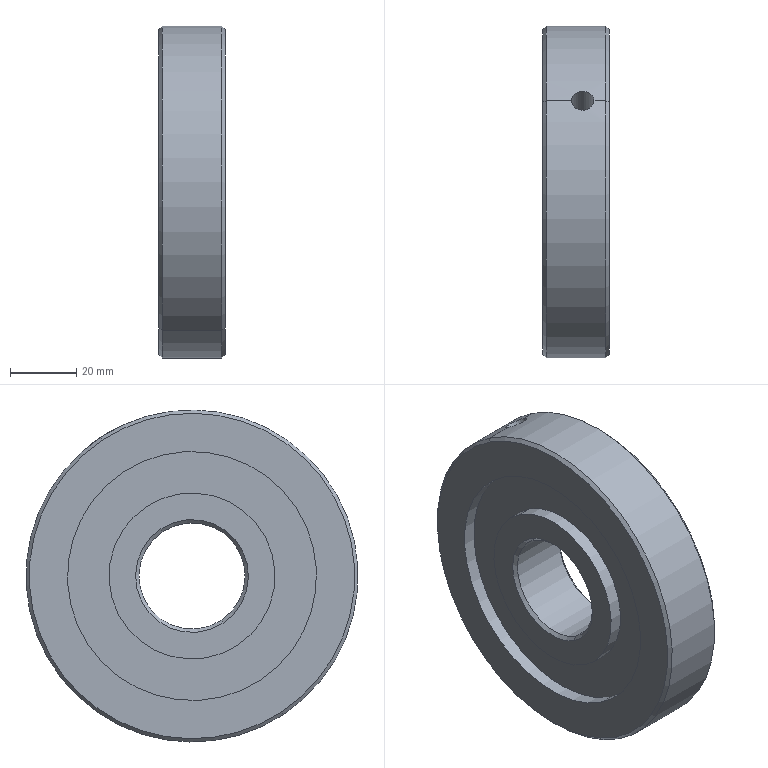Component | SolidWorks | Flange2-1 | 1 solid | 22 faces | box 20 x 100 x 100 mm | volume 129525 mm3 | cylinder 10 | cone 8 | plane 4 | commonest cylinder face diameters 6.8 x2 50 x2 75 x2 32 x2 100 x2
build123d program:
from build123d import *

# Parameters (mm, degrees)
SKETCH1_R             = 50
SKETCH1_R_2           = 16
BOSS_EXTRUDE1_DEPTH   = 20
CHAMFER1_SIZE         = 1
SKETCH2_R             = 37.5
SKETCH2_R_2           = 25
CUT_EXTRUDE1_DEPTH    = 4
M8_TAPPED_HOLE1_D     = 6.8
M8_TAPPED_HOLE1_DEPTH = 41.75
M8_TAPPED_HOLE1_TIP   = 2.043


with BuildPart() as part:
    # Sketch1 → Boss-Extrude1 (new body)
    with BuildSketch(Plane.XY):
        Circle(SKETCH1_R)
        Circle(SKETCH1_R_2, mode=Mode.SUBTRACT)
    extrude(amount=BOSS_EXTRUDE1_DEPTH)

    # Chamfer1
    chamfer1_edges = [part.edges().sort_by_distance(p)[0] for p in [
        (-50, 0, 0),
        (-50, 0, 20),
        (-16, 0, 0),
        (-16, 0, 20),
    ]]
    chamfer(chamfer1_edges, length=CHAMFER1_SIZE)

    # Sketch2 → Cut-Extrude1 (cut)
    with BuildSketch(Plane.XY.offset(20)):
        Circle(SKETCH2_R)
        Circle(SKETCH2_R_2, mode=Mode.SUBTRACT)
    extrude(amount=-CUT_EXTRUDE1_DEPTH, mode=Mode.SUBTRACT)

    # M8 Tapped Hole1
    with Locations(Plane(origin=(50, 0, 8), x_dir=(0, 1, 0), z_dir=(1, 0, 0))):
        with Locations((0, 0)):
            Hole(M8_TAPPED_HOLE1_D / 2, depth=M8_TAPPED_HOLE1_DEPTH)
            with Locations((0, 0, -(M8_TAPPED_HOLE1_DEPTH + M8_TAPPED_HOLE1_TIP / 2))):  # 118° drill point
                Cone(0, M8_TAPPED_HOLE1_D / 2, M8_TAPPED_HOLE1_TIP, mode=Mode.SUBTRACT)


solid = part.part

# Placed as in the assembly
solid = solid.moved(Location((-136.809, -4.181, 0), (-33.315, -90, 0)))
STEP:
#1=COLOUR_RGB('',0.7922,0.8196,0.9333);
#2=FILL_AREA_STYLE_COLOUR('',#1);
#3=FILL_AREA_STYLE('',(#2));
#4=SURFACE_STYLE_FILL_AREA(#3);
#5=SURFACE_SIDE_STYLE('',(#4));
#6=SURFACE_STYLE_USAGE(.BOTH.,#5);
#7=PRESENTATION_STYLE_ASSIGNMENT((#6));
#8=CARTESIAN_POINT('',(-5.567,0.1814,0.5264));
#9=VERTEX_POINT('',#8);
#10=CARTESIAN_POINT('',(-5.835,0.1814,0.5264));
#11=VERTEX_POINT('',#10);
#12=CARTESIAN_POINT('',(-5.567,0.1814,0.5264));
#13=CARTESIAN_POINT('',(-5.567,0.174,0.5313));
#14=CARTESIAN_POINT('',(-5.568,0.1666,0.5359));
#15=CARTESIAN_POINT('',(-5.572,0.1518,0.5447));
#16=CARTESIAN_POINT('',(-5.574,0.1444,0.549));
#17=CARTESIAN_POINT('',(-5.581,0.1302,0.5568));
#18=CARTESIAN_POINT('',(-5.585,0.1233,0.5603));
#19=CARTESIAN_POINT('',(-5.595,0.1102,0.5669));
#20=CARTESIAN_POINT('',(-5.6,0.104,0.5698));
#21=CARTESIAN_POINT('',(-5.613,0.09266,0.575));
#22=CARTESIAN_POINT('',(-5.619,0.08753,0.5773));
#23=CARTESIAN_POINT('',(-5.634,0.07839,0.5812));
#24=CARTESIAN_POINT('',(-5.642,0.07449,0.5828));
#25=CARTESIAN_POINT('',(-5.658,0.06817,0.5853));
#26=CARTESIAN_POINT('',(-5.666,0.06571,0.5863));
#27=CARTESIAN_POINT('',(-5.684,0.06243,0.5876));
#28=CARTESIAN_POINT('',(-5.692,0.06161,0.5879));
#29=CARTESIAN_POINT('',(-5.71,0.0616,0.5879));
#30=CARTESIAN_POINT('',(-5.719,0.06244,0.5876));
#31=CARTESIAN_POINT('',(-5.736,0.06571,0.5863));
#32=CARTESIAN_POINT('',(-5.744,0.06812,0.5854));
#33=CARTESIAN_POINT('',(-5.761,0.07449,0.5828));
#34=CARTESIAN_POINT('',(-5.768,0.07843,0.5812));
#35=CARTESIAN_POINT('',(-5.783,0.08747,0.5773));
#36=CARTESIAN_POINT('',(-5.79,0.09264,0.575));
#37=CARTESIAN_POINT('',(-5.802,0.1041,0.5698));
#38=CARTESIAN_POINT('',(-5.808,0.1102,0.5669));
#39=CARTESIAN_POINT('',(-5.817,0.1232,0.5604));
#40=CARTESIAN_POINT('',(-5.821,0.1302,0.5567));
#41=CARTESIAN_POINT('',(-5.828,0.1445,0.5489));
#42=CARTESIAN_POINT('',(-5.831,0.1517,0.5448));
#43=CARTESIAN_POINT('',(-5.834,0.1665,0.5359));
#44=CARTESIAN_POINT('',(-5.835,0.1741,0.5312));
#45=CARTESIAN_POINT('',(-5.835,0.1814,0.5264));
#46=B_SPLINE_CURVE_WITH_KNOTS('',3,(#12,#13,#14,#15,#16,#17,#18,#19,#20,#21,#22,#23,#24,#25,#26,#27,#28,#29,#30,#31,#32,#33,#34,#35,#36,#37,#38,#39,#40,#41,#42,#43,#44,#45),.UNSPECIFIED.,.F.,.F.,(4,2,2,2,2,2,2,2,2,2,2,2,2,2,2,2,4),(0.,0.0006663,0.001333,0.001999,0.002665,0.003331,0.003998,0.004664,0.00533,0.005996,0.006663,0.007329,0.007995,0.008662,0.009328,0.009994,0.01066),.UNSPECIFIED.);
#47=EDGE_CURVE('',#9,#11,#46,.T.);
#48=ORIENTED_EDGE('',*,*,#47,.T.);
#49=CARTESIAN_POINT('',(-5.835,0.9166,1.645));
#50=VERTEX_POINT('',#49);
#51=CARTESIAN_POINT('',(-5.835,0.9166,1.645));
#52=DIRECTION('',(-0.,0.5492,0.8357));
#53=VECTOR('',#52,39.37);
#54=LINE('',#51,#53);
#55=EDGE_CURVE('',#11,#50,#54,.T.);
#56=ORIENTED_EDGE('',*,*,#55,.T.);
#57=CARTESIAN_POINT('',(-5.567,0.9166,1.645));
#58=VERTEX_POINT('',#57);
#59=CARTESIAN_POINT('',(-5.567,0.9166,1.645));
#60=CARTESIAN_POINT('',(-5.567,0.9092,1.65));
#61=CARTESIAN_POINT('',(-5.568,0.9019,1.655));
#62=CARTESIAN_POINT('',(-5.572,0.8874,1.664));
#63=CARTESIAN_POINT('',(-5.574,0.8802,1.668));
#64=CARTESIAN_POINT('',(-5.581,0.8665,1.677));
#65=CARTESIAN_POINT('',(-5.585,0.8599,1.681));
#66=CARTESIAN_POINT('',(-5.595,0.8474,1.688));
#67=CARTESIAN_POINT('',(-5.6,0.8415,1.692));
#68=CARTESIAN_POINT('',(-5.613,0.8309,1.698));
#69=CARTESIAN_POINT('',(-5.619,0.8261,1.701));
#70=CARTESIAN_POINT('',(-5.634,0.8176,1.706));
#71=CARTESIAN_POINT('',(-5.642,0.814,1.708));
#72=CARTESIAN_POINT('',(-5.658,0.8082,1.711));
#73=CARTESIAN_POINT('',(-5.666,0.8059,1.713));
#74=CARTESIAN_POINT('',(-5.684,0.8029,1.714));
#75=CARTESIAN_POINT('',(-5.692,0.8022,1.715));
#76=CARTESIAN_POINT('',(-5.71,0.8022,1.715));
#77=CARTESIAN_POINT('',(-5.719,0.803,1.714));
#78=CARTESIAN_POINT('',(-5.736,0.8059,1.713));
#79=CARTESIAN_POINT('',(-5.744,0.8081,1.711));
#80=CARTESIAN_POINT('',(-5.76,0.814,1.708));
#81=CARTESIAN_POINT('',(-5.768,0.8176,1.706));
#82=CARTESIAN_POINT('',(-5.783,0.826,1.701));
#83=CARTESIAN_POINT('',(-5.79,0.8308,1.698));
#84=CARTESIAN_POINT('',(-5.802,0.8416,1.692));
#85=CARTESIAN_POINT('',(-5.808,0.8474,1.688));
#86=CARTESIAN_POINT('',(-5.817,0.8598,1.681));
#87=CARTESIAN_POINT('',(-5.821,0.8665,1.677));
#88=CARTESIAN_POINT('',(-5.828,0.8803,1.668));
#89=CARTESIAN_POINT('',(-5.831,0.8874,1.664));
#90=CARTESIAN_POINT('',(-5.834,0.9018,1.655));
#91=CARTESIAN_POINT('',(-5.835,0.9093,1.65));
#92=CARTESIAN_POINT('',(-5.835,0.9166,1.645));
#93=B_SPLINE_CURVE_WITH_KNOTS('',3,(#59,#60,#61,#62,#63,#64,#65,#66,#67,#68,#69,#70,#71,#72,#73,#74,#75,#76,#77,#78,#79,#80,#81,#82,#83,#84,#85,#86,#87,#88,#89,#90,#91,#92),.UNSPECIFIED.,.F.,.F.,(4,2,2,2,2,2,2,2,2,2,2,2,2,2,2,2,4),(0.,0.0006646,0.001329,0.001994,0.002658,0.003323,0.003987,0.004652,0.005317,0.005981,0.006646,0.00731,0.007975,0.008639,0.009304,0.009968,0.01063),.UNSPECIFIED.);
#94=EDGE_CURVE('',#58,#50,#93,.T.);
#95=ORIENTED_EDGE('',*,*,#94,.F.);
#96=CARTESIAN_POINT('',(-5.567,0.9166,1.645));
#97=DIRECTION('',(-0.,0.5492,0.8357));
#98=VECTOR('',#97,39.37);
#99=LINE('',#96,#98);
#100=EDGE_CURVE('',#9,#58,#99,.T.);
#101=ORIENTED_EDGE('',*,*,#100,.F.);
#102=EDGE_LOOP('',(#48,#56,#95,#101));
#103=FACE_OUTER_BOUND('',#102,.T.);
#104=CARTESIAN_POINT('',(-5.701,0.9166,1.645));
#105=DIRECTION('',(-0.,0.5492,0.8357));
#106=DIRECTION('',(1.,0.,0.));
#107=AXIS2_PLACEMENT_3D('',#104,#105,#106);
#108=CYLINDRICAL_SURFACE('',#107,0.1339);
#109=ADVANCED_FACE('',(#103),#108,.F.);
#110=CARTESIAN_POINT('',(-6.016,0.376,0.8225));
#111=VERTEX_POINT('',#110);
#112=CARTESIAN_POINT('',(-6.016,-0.7052,-0.8225));
#113=VERTEX_POINT('',#112);
#114=CARTESIAN_POINT('',(-6.016,-0.1646,-0.));
#115=DIRECTION('',(-1.,-0.,-0.));
#116=DIRECTION('',(0.,0.5492,0.8357));
#117=AXIS2_PLACEMENT_3D('',#114,#115,#116);
#118=CIRCLE('',#117,0.9843);
#119=EDGE_CURVE('',#111,#113,#118,.T.);
#120=ORIENTED_EDGE('',*,*,#119,.T.);
#121=CARTESIAN_POINT('',(-6.174,-0.7052,-0.8225));
#122=VERTEX_POINT('',#121);
#123=CARTESIAN_POINT('',(-6.016,-0.7052,-0.8225));
#124=DIRECTION('',(-1.,-0.,-0.));
#125=VECTOR('',#124,39.37);
#126=LINE('',#123,#125);
#127=EDGE_CURVE('',#113,#122,#126,.T.);
#128=ORIENTED_EDGE('',*,*,#127,.T.);
#129=CARTESIAN_POINT('',(-6.174,0.376,0.8225));
#130=VERTEX_POINT('',#129);
#131=CARTESIAN_POINT('',(-6.174,-0.1646,-0.));
#132=DIRECTION('',(-1.,-0.,-0.));
#133=DIRECTION('',(0.,0.5492,0.8357));
#134=AXIS2_PLACEMENT_3D('',#131,#132,#133);
#135=CIRCLE('',#134,0.9843);
#136=EDGE_CURVE('',#130,#122,#135,.T.);
#137=ORIENTED_EDGE('',*,*,#136,.F.);
#138=CARTESIAN_POINT('',(-6.016,0.376,0.8225));
#139=DIRECTION('',(-1.,-0.,-0.));
#140=VECTOR('',#139,39.37);
#141=LINE('',#138,#140);
#142=EDGE_CURVE('',#111,#130,#141,.T.);
#143=ORIENTED_EDGE('',*,*,#142,.F.);
#144=EDGE_LOOP('',(#120,#128,#137,#143));
#145=FACE_OUTER_BOUND('',#144,.T.);
#146=CARTESIAN_POINT('',(-6.016,-0.1646,-0.));
#147=DIRECTION('',(-1.,-0.,-0.));
#148=DIRECTION('',(0.,0.5492,0.8357));
#149=AXIS2_PLACEMENT_3D('',#146,#147,#148);
#150=CYLINDRICAL_SURFACE('',#149,0.9843);
#151=ADVANCED_FACE('',(#145),#150,.T.);
#152=CARTESIAN_POINT('',(-6.016,-0.9755,-1.234));
#153=VERTEX_POINT('',#152);
#154=CARTESIAN_POINT('',(-6.016,0.6463,1.234));
#155=VERTEX_POINT('',#154);
#156=CARTESIAN_POINT('',(-6.016,-0.1646,-0.));
#157=DIRECTION('',(-1.,-0.,-0.));
#158=DIRECTION('',(0.,0.5492,0.8357));
#159=AXIS2_PLACEMENT_3D('',#156,#157,#158);
#160=CIRCLE('',#159,1.476);
#161=EDGE_CURVE('',#153,#155,#160,.T.);
#162=ORIENTED_EDGE('',*,*,#161,.F.);
#163=CARTESIAN_POINT('',(-6.174,-0.9755,-1.234));
#164=VERTEX_POINT('',#163);
#165=CARTESIAN_POINT('',(-6.016,-0.9755,-1.234));
#166=DIRECTION('',(-1.,-0.,-0.));
#167=VECTOR('',#166,39.37);
#168=LINE('',#165,#167);
#169=EDGE_CURVE('',#153,#164,#168,.T.);
#170=ORIENTED_EDGE('',*,*,#169,.T.);
#171=CARTESIAN_POINT('',(-6.174,0.6463,1.234));
#172=VERTEX_POINT('',#171);
#173=CARTESIAN_POINT('',(-6.174,-0.1646,-0.));
#174=DIRECTION('',(-1.,-0.,-0.));
#175=DIRECTION('',(0.,0.5492,0.8357));
#176=AXIS2_PLACEMENT_3D('',#173,#174,#175);
#177=CIRCLE('',#176,1.476);
#178=EDGE_CURVE('',#164,#172,#177,.T.);
#179=ORIENTED_EDGE('',*,*,#178,.T.);
#180=CARTESIAN_POINT('',(-6.016,0.6463,1.234));
#181=DIRECTION('',(-1.,-0.,-0.));
#182=VECTOR('',#181,39.37);
#183=LINE('',#180,#182);
#184=EDGE_CURVE('',#155,#172,#183,.T.);
#185=ORIENTED_EDGE('',*,*,#184,.F.);
#186=EDGE_LOOP('',(#162,#170,#179,#185));
#187=FACE_OUTER_BOUND('',#186,.T.);
#188=CARTESIAN_POINT('',(-6.016,-0.1646,-0.));
#189=DIRECTION('',(-1.,-0.,-0.));
#190=DIRECTION('',(0.,0.5492,0.8357));
#191=AXIS2_PLACEMENT_3D('',#188,#189,#190);
#192=CYLINDRICAL_SURFACE('',#191,1.476);
#193=ADVANCED_FACE('',(#187),#192,.F.);
#194=CARTESIAN_POINT('',(-6.174,0.8949,1.612));
#195=VERTEX_POINT('',#194);
#196=CARTESIAN_POINT('',(-6.174,-1.224,-1.612));
#197=VERTEX_POINT('',#196);
#198=CARTESIAN_POINT('',(-6.174,-0.1646,-0.));
#199=DIRECTION('',(-1.,-0.,-0.));
#200=DIRECTION('',(0.,0.5492,0.8357));
#201=AXIS2_PLACEMENT_3D('',#198,#199,#200);
#202=CIRCLE('',#201,1.929);
#203=EDGE_CURVE('',#195,#197,#202,.T.);
#204=ORIENTED_EDGE('',*,*,#203,.F.);
#205=CARTESIAN_POINT('',(-6.134,0.9166,1.645));
#206=VERTEX_POINT('',#205);
#207=CARTESIAN_POINT('',(-6.174,0.8949,1.612));
#208=DIRECTION('',(0.7071,0.3884,0.5909));
#209=VECTOR('',#208,39.37);
#210=LINE('',#207,#209);
#211=EDGE_CURVE('',#195,#206,#210,.T.);
#212=ORIENTED_EDGE('',*,*,#211,.T.);
#213=CARTESIAN_POINT('',(-6.134,-1.246,-1.645));
#214=VERTEX_POINT('',#213);
#215=CARTESIAN_POINT('',(-6.134,-0.1646,-0.));
#216=DIRECTION('',(1.,0.,0.));
#217=DIRECTION('',(0.,0.5492,0.8357));
#218=AXIS2_PLACEMENT_3D('',#215,#216,#217);
#219=CIRCLE('',#218,1.969);
#220=EDGE_CURVE('',#214,#206,#219,.T.);
#221=ORIENTED_EDGE('',*,*,#220,.F.);
#222=CARTESIAN_POINT('',(-6.174,-1.224,-1.612));
#223=DIRECTION('',(0.7071,-0.3884,-0.5909));
#224=VECTOR('',#223,39.37);
#225=LINE('',#222,#224);
#226=EDGE_CURVE('',#197,#214,#225,.T.);
#227=ORIENTED_EDGE('',*,*,#226,.F.);
#228=EDGE_LOOP('',(#204,#212,#221,#227));
#229=FACE_OUTER_BOUND('',#228,.T.);
#230=CARTESIAN_POINT('',(-6.174,-0.1646,-0.));
#231=DIRECTION('',(1.,0.,0.));
#232=DIRECTION('',(0.,-0.5492,-0.8357));
#233=AXIS2_PLACEMENT_3D('',#230,#231,#232);
#234=CONICAL_SURFACE('',#233,1.929,0.7854);
#235=ADVANCED_FACE('',(#229),#234,.T.);
#236=CARTESIAN_POINT('',(-6.134,-0.5106,-0.5264));
#237=VERTEX_POINT('',#236);
#238=CARTESIAN_POINT('',(-6.134,0.1814,0.5264));
#239=VERTEX_POINT('',#238);
#240=CARTESIAN_POINT('',(-6.134,-0.1646,-0.));
#241=DIRECTION('',(-1.,-0.,-0.));
#242=DIRECTION('',(0.,0.5492,0.8357));
#243=AXIS2_PLACEMENT_3D('',#240,#241,#242);
#244=CIRCLE('',#243,0.6299);
#245=EDGE_CURVE('',#237,#239,#244,.T.);
#246=ORIENTED_EDGE('',*,*,#245,.F.);
#247=CARTESIAN_POINT('',(-6.174,-0.5322,-0.5593));
#248=VERTEX_POINT('',#247);
#249=CARTESIAN_POINT('',(-6.134,-0.5106,-0.5264));
#250=DIRECTION('',(-0.7071,-0.3884,-0.5909));
#251=VECTOR('',#250,39.37);
#252=LINE('',#249,#251);
#253=EDGE_CURVE('',#237,#248,#252,.T.);
#254=ORIENTED_EDGE('',*,*,#253,.T.);
#255=CARTESIAN_POINT('',(-6.174,0.203,0.5593));
#256=VERTEX_POINT('',#255);
#257=CARTESIAN_POINT('',(-6.174,-0.1646,-0.));
#258=DIRECTION('',(1.,0.,0.));
#259=DIRECTION('',(0.,0.5492,0.8357));
#260=AXIS2_PLACEMENT_3D('',#257,#258,#259);
#261=CIRCLE('',#260,0.6693);
#262=EDGE_CURVE('',#256,#248,#261,.T.);
#263=ORIENTED_EDGE('',*,*,#262,.F.);
#264=CARTESIAN_POINT('',(-6.134,0.1814,0.5264));
#265=DIRECTION('',(-0.7071,0.3884,0.5909));
#266=VECTOR('',#265,39.37);
#267=LINE('',#264,#266);
#268=EDGE_CURVE('',#239,#256,#267,.T.);
#269=ORIENTED_EDGE('',*,*,#268,.F.);
#270=EDGE_LOOP('',(#246,#254,#263,#269));
#271=FACE_OUTER_BOUND('',#270,.T.);
#272=CARTESIAN_POINT('',(-6.134,-0.1646,-0.));
#273=DIRECTION('',(-1.,-0.,-0.));
#274=DIRECTION('',(0.,0.5492,0.8357));
#275=AXIS2_PLACEMENT_3D('',#272,#273,#274);
#276=CONICAL_SURFACE('',#275,0.6299,0.7854);
#277=ADVANCED_FACE('',(#271),#276,.F.);
#278=CARTESIAN_POINT('',(-5.386,-1.224,-1.612));
#279=VERTEX_POINT('',#278);
#280=CARTESIAN_POINT('',(-5.386,0.8949,1.612));
#281=VERTEX_POINT('',#280);
#282=CARTESIAN_POINT('',(-5.386,-0.1646,0.));
#283=DIRECTION('',(1.,0.,0.));
#284=DIRECTION('',(0.,0.5492,0.8357));
#285=AXIS2_PLACEMENT_3D('',#282,#283,#284);
#286=CIRCLE('',#285,1.929);
#287=EDGE_CURVE('',#279,#281,#286,.T.);
#288=ORIENTED_EDGE('',*,*,#287,.F.);
#289=CARTESIAN_POINT('',(-5.426,-1.246,-1.645));
#290=VERTEX_POINT('',#289);
#291=CARTESIAN_POINT('',(-5.426,-1.246,-1.645));
#292=DIRECTION('',(-0.7071,-0.3884,-0.5909));
#293=VECTOR('',#292,39.37);
#294=LINE('',#291,#293);
#295=EDGE_CURVE('',#279,#290,#294,.T.);
#296=ORIENTED_EDGE('',*,*,#295,.T.);
#297=CARTESIAN_POINT('',(-5.426,0.9166,1.645));
#298=VERTEX_POINT('',#297);
#299=CARTESIAN_POINT('',(-5.426,-0.1646,0.));
#300=DIRECTION('',(-1.,-0.,-0.));
#301=DIRECTION('',(0.,0.5492,0.8357));
#302=AXIS2_PLACEMENT_3D('',#299,#300,#301);
#303=CIRCLE('',#302,1.969);
#304=EDGE_CURVE('',#298,#290,#303,.T.);
#305=ORIENTED_EDGE('',*,*,#304,.F.);
#306=CARTESIAN_POINT('',(-5.426,0.9166,1.645));
#307=DIRECTION('',(-0.7071,0.3884,0.5909));
#308=VECTOR('',#307,39.37);
#309=LINE('',#306,#308);
#310=EDGE_CURVE('',#281,#298,#309,.T.);
#311=ORIENTED_EDGE('',*,*,#310,.F.);
#312=EDGE_LOOP('',(#288,#296,#305,#311));
#313=FACE_OUTER_BOUND('',#312,.T.);
#314=CARTESIAN_POINT('',(-5.426,-0.1646,0.));
#315=DIRECTION('',(-1.,-0.,-0.));
#316=DIRECTION('',(0.,0.5492,0.8357));
#317=AXIS2_PLACEMENT_3D('',#314,#315,#316);
#318=CONICAL_SURFACE('',#317,1.969,0.7854);
#319=ADVANCED_FACE('',(#313),#318,.T.);
#320=CARTESIAN_POINT('',(-5.426,0.1814,0.5264));
#321=VERTEX_POINT('',#320);
#322=CARTESIAN_POINT('',(-5.426,-0.5106,-0.5264));
#323=VERTEX_POINT('',#322);
#324=CARTESIAN_POINT('',(-5.426,-0.1646,0.));
#325=DIRECTION('',(1.,0.,0.));
#326=DIRECTION('',(0.,0.5492,0.8357));
#327=AXIS2_PLACEMENT_3D('',#324,#325,#326);
#328=CIRCLE('',#327,0.6299);
#329=EDGE_CURVE('',#321,#323,#328,.T.);
#330=ORIENTED_EDGE('',*,*,#329,.F.);
#331=CARTESIAN_POINT('',(-5.386,0.203,0.5593));
#332=VERTEX_POINT('',#331);
#333=CARTESIAN_POINT('',(-5.386,0.203,0.5593));
#334=DIRECTION('',(0.7071,0.3884,0.5909));
#335=VECTOR('',#334,39.37);
#336=LINE('',#333,#335);
#337=EDGE_CURVE('',#321,#332,#336,.T.);
#338=ORIENTED_EDGE('',*,*,#337,.T.);
#339=CARTESIAN_POINT('',(-5.386,-0.5322,-0.5593));
#340=VERTEX_POINT('',#339);
#341=CARTESIAN_POINT('',(-5.386,-0.1646,0.));
#342=DIRECTION('',(-1.,-0.,-0.));
#343=DIRECTION('',(0.,0.5492,0.8357));
#344=AXIS2_PLACEMENT_3D('',#341,#342,#343);
#345=CIRCLE('',#344,0.6693);
#346=EDGE_CURVE('',#340,#332,#345,.T.);
#347=ORIENTED_EDGE('',*,*,#346,.F.);
#348=CARTESIAN_POINT('',(-5.386,-0.5322,-0.5593));
#349=DIRECTION('',(0.7071,-0.3884,-0.5909));
#350=VECTOR('',#349,39.37);
#351=LINE('',#348,#350);
#352=EDGE_CURVE('',#323,#340,#351,.T.);
#353=ORIENTED_EDGE('',*,*,#352,.F.);
#354=EDGE_LOOP('',(#330,#338,#347,#353));
#355=FACE_OUTER_BOUND('',#354,.T.);
#356=CARTESIAN_POINT('',(-5.386,-0.1646,0.));
#357=DIRECTION('',(1.,0.,0.));
#358=DIRECTION('',(0.,-0.5492,-0.8357));
#359=AXIS2_PLACEMENT_3D('',#356,#357,#358);
#360=CONICAL_SURFACE('',#359,0.6693,0.7854);
#361=ADVANCED_FACE('',(#355),#360,.F.);
#362=ORIENTED_EDGE('',*,*,#245,.T.);
#363=CARTESIAN_POINT('',(-6.174,0.1814,0.5264));
#364=DIRECTION('',(1.,0.,0.));
#365=VECTOR('',#364,39.37);
#366=LINE('',#363,#365);
#367=EDGE_CURVE('',#239,#11,#366,.T.);
#368=ORIENTED_EDGE('',*,*,#367,.T.);
#369=ORIENTED_EDGE('',*,*,#47,.F.);
#370=CARTESIAN_POINT('',(-6.174,0.1814,0.5264));
#371=DIRECTION('',(1.,0.,0.));
#372=VECTOR('',#371,39.37);
#373=LINE('',#370,#372);
#374=EDGE_CURVE('',#9,#321,#373,.T.);
#375=ORIENTED_EDGE('',*,*,#374,.T.);
#376=ORIENTED_EDGE('',*,*,#329,.T.);
#377=CARTESIAN_POINT('',(-6.174,-0.5106,-0.5264));
#378=DIRECTION('',(1.,0.,0.));
#379=VECTOR('',#378,39.37);
#380=LINE('',#377,#379);
#381=EDGE_CURVE('',#237,#323,#380,.T.);
#382=ORIENTED_EDGE('',*,*,#381,.F.);
#383=EDGE_LOOP('',(#362,#368,#369,#375,#376,#382));
#384=FACE_OUTER_BOUND('',#383,.T.);
#385=CARTESIAN_POINT('',(-6.174,-0.1646,-0.));
#386=DIRECTION('',(1.,0.,0.));
#387=DIRECTION('',(0.,-0.5492,-0.8357));
#388=AXIS2_PLACEMENT_3D('',#385,#386,#387);
#389=CYLINDRICAL_SURFACE('',#388,0.6299);
#390=ADVANCED_FACE('',(#384),#389,.F.);
#391=ORIENTED_EDGE('',*,*,#220,.T.);
#392=CARTESIAN_POINT('',(-6.174,0.9166,1.645));
#393=DIRECTION('',(1.,0.,0.));
#394=VECTOR('',#393,39.37);
#395=LINE('',#392,#394);
#396=EDGE_CURVE('',#206,#50,#395,.T.);
#397=ORIENTED_EDGE('',*,*,#396,.T.);
#398=CARTESIAN_POINT('',(-5.835,0.9166,1.645));
#399=CARTESIAN_POINT('',(-5.835,0.9239,1.64));
#400=CARTESIAN_POINT('',(-5.834,0.9311,1.635));
#401=CARTESIAN_POINT('',(-5.831,0.9454,1.626));
#402=CARTESIAN_POINT('',(-5.828,0.9524,1.621));
#403=CARTESIAN_POINT('',(-5.821,0.9656,1.612));
#404=CARTESIAN_POINT('',(-5.817,0.972,1.607));
#405=CARTESIAN_POINT('',(-5.808,0.9839,1.599));
#406=CARTESIAN_POINT('',(-5.802,0.9894,1.595));
#407=CARTESIAN_POINT('',(-5.79,0.9994,1.588));
#408=CARTESIAN_POINT('',(-5.783,1.004,1.584));
#409=CARTESIAN_POINT('',(-5.768,1.012,1.578));
#410=CARTESIAN_POINT('',(-5.761,1.015,1.576));
#411=CARTESIAN_POINT('',(-5.744,1.02,1.572));
#412=CARTESIAN_POINT('',(-5.736,1.022,1.57));
#413=CARTESIAN_POINT('',(-5.719,1.025,1.568));
#414=CARTESIAN_POINT('',(-5.71,1.026,1.568));
#415=CARTESIAN_POINT('',(-5.692,1.026,1.568));
#416=CARTESIAN_POINT('',(-5.684,1.025,1.568));
#417=CARTESIAN_POINT('',(-5.667,1.023,1.57));
#418=CARTESIAN_POINT('',(-5.658,1.02,1.572));
#419=CARTESIAN_POINT('',(-5.642,1.015,1.576));
#420=CARTESIAN_POINT('',(-5.634,1.012,1.578));
#421=CARTESIAN_POINT('',(-5.62,1.004,1.584));
#422=CARTESIAN_POINT('',(-5.613,0.9995,1.587));
#423=CARTESIAN_POINT('',(-5.6,0.9895,1.595));
#424=CARTESIAN_POINT('',(-5.595,0.984,1.599));
#425=CARTESIAN_POINT('',(-5.585,0.9721,1.607));
#426=CARTESIAN_POINT('',(-5.581,0.9657,1.612));
#427=CARTESIAN_POINT('',(-5.571,0.9459,1.625));
#428=CARTESIAN_POINT('',(-5.567,0.9313,1.635));
#429=CARTESIAN_POINT('',(-5.567,0.9166,1.645));
#430=B_SPLINE_CURVE_WITH_KNOTS('',3,(#398,#399,#400,#401,#402,#403,#404,#405,#406,#407,#408,#409,#410,#411,#412,#413,#414,#415,#416,#417,#418,#419,#420,#421,#422,#423,#424,#425,#426,#427,#428,#429),.UNSPECIFIED.,.F.,.F.,(4,2,2,2,2,2,2,2,2,2,2,2,2,2,2,4),(0.01063,0.0113,0.01196,0.01263,0.01329,0.01396,0.01462,0.01528,0.01595,0.01661,0.01728,0.01794,0.01861,0.01927,0.01993,0.02126),.UNSPECIFIED.);
#431=EDGE_CURVE('',#50,#58,#430,.T.);
#432=ORIENTED_EDGE('',*,*,#431,.T.);
#433=CARTESIAN_POINT('',(-6.174,0.9166,1.645));
#434=DIRECTION('',(1.,0.,0.));
#435=VECTOR('',#434,39.37);
#436=LINE('',#433,#435);
#437=EDGE_CURVE('',#58,#298,#436,.T.);
#438=ORIENTED_EDGE('',*,*,#437,.T.);
#439=ORIENTED_EDGE('',*,*,#304,.T.);
#440=CARTESIAN_POINT('',(-6.174,-1.246,-1.645));
#441=DIRECTION('',(1.,0.,0.));
#442=VECTOR('',#441,39.37);
#443=LINE('',#440,#442);
#444=EDGE_CURVE('',#214,#290,#443,.T.);
#445=ORIENTED_EDGE('',*,*,#444,.F.);
#446=EDGE_LOOP('',(#391,#397,#432,#438,#439,#445));
#447=FACE_OUTER_BOUND('',#446,.T.);
#448=CARTESIAN_POINT('',(-6.174,-0.1646,-0.));
#449=DIRECTION('',(1.,0.,0.));
#450=DIRECTION('',(0.,-0.5492,-0.8357));
#451=AXIS2_PLACEMENT_3D('',#448,#449,#450);
#452=CYLINDRICAL_SURFACE('',#451,1.969);
#453=ADVANCED_FACE('',(#447),#452,.T.);
#454=ORIENTED_EDGE('',*,*,#262,.T.);
#455=CARTESIAN_POINT('',(-6.174,-0.1646,-0.));
#456=DIRECTION('',(1.,0.,0.));
#457=DIRECTION('',(0.,0.5492,0.8357));
#458=AXIS2_PLACEMENT_3D('',#455,#456,#457);
#459=CIRCLE('',#458,0.6693);
#460=EDGE_CURVE('',#248,#256,#459,.T.);
#461=ORIENTED_EDGE('',*,*,#460,.T.);
#462=EDGE_LOOP('',(#454,#461));
#463=FACE_BOUND('',#462,.T.);
#464=ORIENTED_EDGE('',*,*,#136,.T.);
#465=CARTESIAN_POINT('',(-6.174,-0.1646,-0.));
#466=DIRECTION('',(-1.,-0.,-0.));
#467=DIRECTION('',(0.,0.5492,0.8357));
#468=AXIS2_PLACEMENT_3D('',#465,#466,#467);
#469=CIRCLE('',#468,0.9843);
#470=EDGE_CURVE('',#122,#130,#469,.T.);
#471=ORIENTED_EDGE('',*,*,#470,.T.);
#472=EDGE_LOOP('',(#464,#471));
#473=FACE_OUTER_BOUND('',#472,.T.);
#474=CARTESIAN_POINT('',(-6.174,-0.1646,-0.));
#475=DIRECTION('',(-1.,-0.,-0.));
#476=DIRECTION('',(-0.,0.5492,0.8357));
#477=AXIS2_PLACEMENT_3D('',#474,#475,#476);
#478=PLANE('',#477);
#479=ADVANCED_FACE('',(#463,#473),#478,.T.);
#480=CARTESIAN_POINT('',(-6.174,-0.1646,-0.));
#481=DIRECTION('',(-1.,-0.,-0.));
#482=DIRECTION('',(0.,0.5492,0.8357));
#483=AXIS2_PLACEMENT_3D('',#480,#481,#482);
#484=CIRCLE('',#483,1.476);
#485=EDGE_CURVE('',#172,#164,#484,.T.);
#486=ORIENTED_EDGE('',*,*,#485,.F.);
#487=ORIENTED_EDGE('',*,*,#178,.F.);
#488=EDGE_LOOP('',(#486,#487));
#489=FACE_BOUND('',#488,.T.);
#490=CARTESIAN_POINT('',(-6.174,-0.1646,-0.));
#491=DIRECTION('',(-1.,-0.,-0.));
#492=DIRECTION('',(0.,0.5492,0.8357));
#493=AXIS2_PLACEMENT_3D('',#490,#491,#492);
#494=CIRCLE('',#493,1.929);
#495=EDGE_CURVE('',#197,#195,#494,.T.);
#496=ORIENTED_EDGE('',*,*,#495,.T.);
#497=ORIENTED_EDGE('',*,*,#203,.T.);
#498=EDGE_LOOP('',(#496,#497));
#499=FACE_OUTER_BOUND('',#498,.T.);
#500=CARTESIAN_POINT('',(-6.174,-0.1646,-0.));
#501=DIRECTION('',(-1.,-0.,-0.));
#502=DIRECTION('',(-0.,0.5492,0.8357));
#503=AXIS2_PLACEMENT_3D('',#500,#501,#502);
#504=PLANE('',#503);
#505=ADVANCED_FACE('',(#489,#499),#504,.T.);
#506=ORIENTED_EDGE('',*,*,#346,.T.);
#507=CARTESIAN_POINT('',(-5.386,-0.1646,0.));
#508=DIRECTION('',(-1.,-0.,-0.));
#509=DIRECTION('',(0.,0.5492,0.8357));
#510=AXIS2_PLACEMENT_3D('',#507,#508,#509);
#511=CIRCLE('',#510,0.6693);
#512=EDGE_CURVE('',#332,#340,#511,.T.);
#513=ORIENTED_EDGE('',*,*,#512,.T.);
#514=EDGE_LOOP('',(#506,#513));
#515=FACE_BOUND('',#514,.T.);
#516=CARTESIAN_POINT('',(-5.386,-0.1646,0.));
#517=DIRECTION('',(1.,0.,0.));
#518=DIRECTION('',(0.,0.5492,0.8357));
#519=AXIS2_PLACEMENT_3D('',#516,#517,#518);
#520=CIRCLE('',#519,1.929);
#521=EDGE_CURVE('',#281,#279,#520,.T.);
#522=ORIENTED_EDGE('',*,*,#521,.T.);
#523=ORIENTED_EDGE('',*,*,#287,.T.);
#524=EDGE_LOOP('',(#522,#523));
#525=FACE_OUTER_BOUND('',#524,.T.);
#526=CARTESIAN_POINT('',(-5.386,-0.1646,0.));
#527=DIRECTION('',(-1.,-0.,-0.));
#528=DIRECTION('',(-0.,0.5492,0.8357));
#529=AXIS2_PLACEMENT_3D('',#526,#527,#528);
#530=PLANE('',#529);
#531=ADVANCED_FACE('',(#515,#525),#530,.F.);
#532=ORIENTED_EDGE('',*,*,#396,.F.);
#533=CARTESIAN_POINT('',(-6.134,-0.1646,-0.));
#534=DIRECTION('',(1.,0.,0.));
#535=DIRECTION('',(0.,0.5492,0.8357));
#536=AXIS2_PLACEMENT_3D('',#533,#534,#535);
#537=CIRCLE('',#536,1.969);
#538=EDGE_CURVE('',#206,#214,#537,.T.);
#539=ORIENTED_EDGE('',*,*,#538,.T.);
#540=ORIENTED_EDGE('',*,*,#444,.T.);
#541=CARTESIAN_POINT('',(-5.426,-0.1646,0.));
#542=DIRECTION('',(-1.,-0.,-0.));
#543=DIRECTION('',(0.,0.5492,0.8357));
#544=AXIS2_PLACEMENT_3D('',#541,#542,#543);
#545=CIRCLE('',#544,1.969);
#546=EDGE_CURVE('',#290,#298,#545,.T.);
#547=ORIENTED_EDGE('',*,*,#546,.T.);
#548=ORIENTED_EDGE('',*,*,#437,.F.);
#549=ORIENTED_EDGE('',*,*,#94,.T.);
#550=EDGE_LOOP('',(#532,#539,#540,#547,#548,#549));
#551=FACE_OUTER_BOUND('',#550,.T.);
#552=CARTESIAN_POINT('',(-6.174,-0.1646,-0.));
#553=DIRECTION('',(1.,0.,0.));
#554=DIRECTION('',(0.,-0.5492,-0.8357));
#555=AXIS2_PLACEMENT_3D('',#552,#553,#554);
#556=CYLINDRICAL_SURFACE('',#555,1.969);
#557=ADVANCED_FACE('',(#551),#556,.T.);
#558=ORIENTED_EDGE('',*,*,#367,.F.);
#559=CARTESIAN_POINT('',(-6.134,-0.1646,-0.));
#560=DIRECTION('',(-1.,-0.,-0.));
#561=DIRECTION('',(0.,0.5492,0.8357));
#562=AXIS2_PLACEMENT_3D('',#559,#560,#561);
#563=CIRCLE('',#562,0.6299);
#564=EDGE_CURVE('',#239,#237,#563,.T.);
#565=ORIENTED_EDGE('',*,*,#564,.T.);
#566=ORIENTED_EDGE('',*,*,#381,.T.);
#567=CARTESIAN_POINT('',(-5.426,-0.1646,0.));
#568=DIRECTION('',(1.,0.,0.));
#569=DIRECTION('',(0.,0.5492,0.8357));
#570=AXIS2_PLACEMENT_3D('',#567,#568,#569);
#571=CIRCLE('',#570,0.6299);
#572=EDGE_CURVE('',#323,#321,#571,.T.);
#573=ORIENTED_EDGE('',*,*,#572,.T.);
#574=ORIENTED_EDGE('',*,*,#374,.F.);
#575=CARTESIAN_POINT('',(-5.835,0.1814,0.5264));
#576=CARTESIAN_POINT('',(-5.835,0.1887,0.5216));
#577=CARTESIAN_POINT('',(-5.834,0.1959,0.5167));
#578=CARTESIAN_POINT('',(-5.831,0.21,0.5065));
#579=CARTESIAN_POINT('',(-5.828,0.2167,0.5015));
#580=CARTESIAN_POINT('',(-5.821,0.2294,0.4915));
#581=CARTESIAN_POINT('',(-5.817,0.2355,0.4866));
#582=CARTESIAN_POINT('',(-5.808,0.2468,0.4771));
#583=CARTESIAN_POINT('',(-5.802,0.2519,0.4726));
#584=CARTESIAN_POINT('',(-5.79,0.2611,0.4643));
#585=CARTESIAN_POINT('',(-5.783,0.2653,0.4604));
#586=CARTESIAN_POINT('',(-5.768,0.2725,0.4536));
#587=CARTESIAN_POINT('',(-5.761,0.2755,0.4507));
#588=CARTESIAN_POINT('',(-5.736,0.2828,0.4434));
#589=CARTESIAN_POINT('',(-5.719,0.2853,0.4409));
#590=CARTESIAN_POINT('',(-5.692,0.2853,0.4409));
#591=CARTESIAN_POINT('',(-5.684,0.2847,0.4415));
#592=CARTESIAN_POINT('',(-5.666,0.2823,0.444));
#593=CARTESIAN_POINT('',(-5.658,0.2804,0.4458));
#594=CARTESIAN_POINT('',(-5.642,0.2755,0.4506));
#595=CARTESIAN_POINT('',(-5.634,0.2725,0.4536));
#596=CARTESIAN_POINT('',(-5.62,0.2654,0.4604));
#597=CARTESIAN_POINT('',(-5.613,0.2612,0.4642));
#598=CARTESIAN_POINT('',(-5.6,0.252,0.4726));
#599=CARTESIAN_POINT('',(-5.595,0.2468,0.477));
#600=CARTESIAN_POINT('',(-5.585,0.2356,0.4865));
#601=CARTESIAN_POINT('',(-5.581,0.2296,0.4914));
#602=CARTESIAN_POINT('',(-5.574,0.2168,0.5014));
#603=CARTESIAN_POINT('',(-5.572,0.21,0.5065));
#604=CARTESIAN_POINT('',(-5.568,0.196,0.5166));
#605=CARTESIAN_POINT('',(-5.567,0.1888,0.5215));
#606=CARTESIAN_POINT('',(-5.567,0.1814,0.5264));
#607=B_SPLINE_CURVE_WITH_KNOTS('',3,(#575,#576,#577,#578,#579,#580,#581,#582,#583,#584,#585,#586,#587,#588,#589,#590,#591,#592,#593,#594,#595,#596,#597,#598,#599,#600,#601,#602,#603,#604,#605,#606),.UNSPECIFIED.,.F.,.F.,(4,2,2,2,2,2,2,2,2,2,2,2,2,2,2,4),(0.01066,0.01133,0.01199,0.01266,0.01332,0.01399,0.01466,0.01599,0.01666,0.01732,0.01799,0.01865,0.01932,0.01999,0.02065,0.02132),.UNSPECIFIED.);
#608=EDGE_CURVE('',#11,#9,#607,.T.);
#609=ORIENTED_EDGE('',*,*,#608,.F.);
#610=EDGE_LOOP('',(#558,#565,#566,#573,#574,#609));
#611=FACE_OUTER_BOUND('',#610,.T.);
#612=CARTESIAN_POINT('',(-6.174,-0.1646,-0.));
#613=DIRECTION('',(1.,0.,0.));
#614=DIRECTION('',(0.,-0.5492,-0.8357));
#615=AXIS2_PLACEMENT_3D('',#612,#613,#614);
#616=CYLINDRICAL_SURFACE('',#615,0.6299);
#617=ADVANCED_FACE('',(#611),#616,.F.);
#618=ORIENTED_EDGE('',*,*,#337,.F.);
#619=ORIENTED_EDGE('',*,*,#572,.F.);
#620=ORIENTED_EDGE('',*,*,#352,.T.);
#621=ORIENTED_EDGE('',*,*,#512,.F.);
#622=EDGE_LOOP('',(#618,#619,#620,#621));
#623=FACE_OUTER_BOUND('',#622,.T.);
#624=CARTESIAN_POINT('',(-5.386,-0.1646,0.));
#625=DIRECTION('',(1.,0.,0.));
#626=DIRECTION('',(0.,-0.5492,-0.8357));
#627=AXIS2_PLACEMENT_3D('',#624,#625,#626);
#628=CONICAL_SURFACE('',#627,0.6693,0.7854);
#629=ADVANCED_FACE('',(#623),#628,.F.);
#630=ORIENTED_EDGE('',*,*,#295,.F.);
#631=ORIENTED_EDGE('',*,*,#521,.F.);
#632=ORIENTED_EDGE('',*,*,#310,.T.);
#633=ORIENTED_EDGE('',*,*,#546,.F.);
#634=EDGE_LOOP('',(#630,#631,#632,#633));
#635=FACE_OUTER_BOUND('',#634,.T.);
#636=CARTESIAN_POINT('',(-5.426,-0.1646,0.));
#637=DIRECTION('',(-1.,-0.,-0.));
#638=DIRECTION('',(0.,0.5492,0.8357));
#639=AXIS2_PLACEMENT_3D('',#636,#637,#638);
#640=CONICAL_SURFACE('',#639,1.969,0.7854);
#641=ADVANCED_FACE('',(#635),#640,.T.);
#642=ORIENTED_EDGE('',*,*,#253,.F.);
#643=ORIENTED_EDGE('',*,*,#564,.F.);
#644=ORIENTED_EDGE('',*,*,#268,.T.);
#645=ORIENTED_EDGE('',*,*,#460,.F.);
#646=EDGE_LOOP('',(#642,#643,#644,#645));
#647=FACE_OUTER_BOUND('',#646,.T.);
#648=CARTESIAN_POINT('',(-6.134,-0.1646,-0.));
#649=DIRECTION('',(-1.,-0.,-0.));
#650=DIRECTION('',(0.,0.5492,0.8357));
#651=AXIS2_PLACEMENT_3D('',#648,#649,#650);
#652=CONICAL_SURFACE('',#651,0.6299,0.7854);
#653=ADVANCED_FACE('',(#647),#652,.F.);
#654=ORIENTED_EDGE('',*,*,#211,.F.);
#655=ORIENTED_EDGE('',*,*,#495,.F.);
#656=ORIENTED_EDGE('',*,*,#226,.T.);
#657=ORIENTED_EDGE('',*,*,#538,.F.);
#658=EDGE_LOOP('',(#654,#655,#656,#657));
#659=FACE_OUTER_BOUND('',#658,.T.);
#660=CARTESIAN_POINT('',(-6.174,-0.1646,-0.));
#661=DIRECTION('',(1.,0.,0.));
#662=DIRECTION('',(0.,-0.5492,-0.8357));
#663=AXIS2_PLACEMENT_3D('',#660,#661,#662);
#664=CONICAL_SURFACE('',#663,1.929,0.7854);
#665=ADVANCED_FACE('',(#659),#664,.T.);
#666=ORIENTED_EDGE('',*,*,#169,.F.);
#667=CARTESIAN_POINT('',(-6.016,-0.1646,-0.));
#668=DIRECTION('',(-1.,-0.,-0.));
#669=DIRECTION('',(0.,0.5492,0.8357));
#670=AXIS2_PLACEMENT_3D('',#667,#668,#669);
#671=CIRCLE('',#670,1.476);
#672=EDGE_CURVE('',#155,#153,#671,.T.);
#673=ORIENTED_EDGE('',*,*,#672,.F.);
#674=ORIENTED_EDGE('',*,*,#184,.T.);
#675=ORIENTED_EDGE('',*,*,#485,.T.);
#676=EDGE_LOOP('',(#666,#673,#674,#675));
#677=FACE_OUTER_BOUND('',#676,.T.);
#678=CARTESIAN_POINT('',(-6.016,-0.1646,-0.));
#679=DIRECTION('',(-1.,-0.,-0.));
#680=DIRECTION('',(0.,0.5492,0.8357));
#681=AXIS2_PLACEMENT_3D('',#678,#679,#680);
#682=CYLINDRICAL_SURFACE('',#681,1.476);
#683=ADVANCED_FACE('',(#677),#682,.F.);
#684=ORIENTED_EDGE('',*,*,#119,.F.);
#685=CARTESIAN_POINT('',(-6.016,-0.1646,-0.));
#686=DIRECTION('',(-1.,-0.,-0.));
#687=DIRECTION('',(0.,0.5492,0.8357));
#688=AXIS2_PLACEMENT_3D('',#685,#686,#687);
#689=CIRCLE('',#688,0.9843);
#690=EDGE_CURVE('',#113,#111,#689,.T.);
#691=ORIENTED_EDGE('',*,*,#690,.F.);
#692=EDGE_LOOP('',(#684,#691));
#693=FACE_BOUND('',#692,.T.);
#694=ORIENTED_EDGE('',*,*,#672,.T.);
#695=ORIENTED_EDGE('',*,*,#161,.T.);
#696=EDGE_LOOP('',(#694,#695));
#697=FACE_OUTER_BOUND('',#696,.T.);
#698=CARTESIAN_POINT('',(-6.016,-0.1646,-0.));
#699=DIRECTION('',(-1.,-0.,-0.));
#700=DIRECTION('',(-0.,0.5492,0.8357));
#701=AXIS2_PLACEMENT_3D('',#698,#699,#700);
#702=PLANE('',#701);
#703=ADVANCED_FACE('',(#693,#697),#702,.T.);
#704=ORIENTED_EDGE('',*,*,#127,.F.);
#705=ORIENTED_EDGE('',*,*,#690,.T.);
#706=ORIENTED_EDGE('',*,*,#142,.T.);
#707=ORIENTED_EDGE('',*,*,#470,.F.);
#708=EDGE_LOOP('',(#704,#705,#706,#707));
#709=FACE_OUTER_BOUND('',#708,.T.);
#710=CARTESIAN_POINT('',(-6.016,-0.1646,-0.));
#711=DIRECTION('',(-1.,-0.,-0.));
#712=DIRECTION('',(0.,0.5492,0.8357));
#713=AXIS2_PLACEMENT_3D('',#710,#711,#712);
#714=CYLINDRICAL_SURFACE('',#713,0.9843);
#715=ADVANCED_FACE('',(#709),#714,.T.);
#716=ORIENTED_EDGE('',*,*,#55,.F.);
#717=ORIENTED_EDGE('',*,*,#608,.T.);
#718=ORIENTED_EDGE('',*,*,#100,.T.);
#719=ORIENTED_EDGE('',*,*,#431,.F.);
#720=EDGE_LOOP('',(#716,#717,#718,#719));
#721=FACE_OUTER_BOUND('',#720,.T.);
#722=CARTESIAN_POINT('',(-5.701,0.9166,1.645));
#723=DIRECTION('',(-0.,0.5492,0.8357));
#724=DIRECTION('',(1.,0.,0.));
#725=AXIS2_PLACEMENT_3D('',#722,#723,#724);
#726=CYLINDRICAL_SURFACE('',#725,0.1339);
#727=ADVANCED_FACE('',(#721),#726,.F.);
#728=CLOSED_SHELL('',(#109,#151,#193,#235,#277,#319,#361,#390,#453,#479,#505,#531,#557,#617,#629,#641,#653,#665,#683,#703,#715,#727));
#729=MANIFOLD_SOLID_BREP('',#728);
#730=STYLED_ITEM('',(#7),#729);
#731=(LENGTH_UNIT()NAMED_UNIT(*)SI_UNIT($,.METRE.));
#732=LENGTH_MEASURE_WITH_UNIT(LENGTH_MEASURE(0.0254),#731);
#733=DIMENSIONAL_EXPONENTS(1.,0.,0.,0.,0.,0.,0.);
#734=(CONVERSION_BASED_UNIT('',#732)LENGTH_UNIT()NAMED_UNIT(#733));
#735=UNCERTAINTY_MEASURE_WITH_UNIT(LENGTH_MEASURE(0.00001),#734,'','');
#736=(NAMED_UNIT(*)PLANE_ANGLE_UNIT()SI_UNIT($,.RADIAN.));
#737=(NAMED_UNIT(*)SI_UNIT($,.STERADIAN.)SOLID_ANGLE_UNIT());
#738=(GEOMETRIC_REPRESENTATION_CONTEXT(3)GLOBAL_UNCERTAINTY_ASSIGNED_CONTEXT((#735))GLOBAL_UNIT_ASSIGNED_CONTEXT((#734,#736,#737))REPRESENTATION_CONTEXT('',''));
#739=MECHANICAL_DESIGN_GEOMETRIC_PRESENTATION_REPRESENTATION('',(#730),#738);
#740=PRESENTATION_LAYER_ASSIGNMENT('','',(#730));
#741=CARTESIAN_POINT('',(0.,0.,0.));
#742=DIRECTION('',(0.,0.,1.));
#743=DIRECTION('',(1.,0.,0.));
#744=AXIS2_PLACEMENT_3D('',#741,#742,#743);
#745=(LENGTH_UNIT()NAMED_UNIT(*)SI_UNIT($,.METRE.));
#746=LENGTH_MEASURE_WITH_UNIT(LENGTH_MEASURE(0.0254),#745);
#747=DIMENSIONAL_EXPONENTS(1.,0.,0.,0.,0.,0.,0.);
#748=(CONVERSION_BASED_UNIT('',#746)LENGTH_UNIT()NAMED_UNIT(#747));
#749=UNCERTAINTY_MEASURE_WITH_UNIT(LENGTH_MEASURE(0.00001),#748,'','');
#750=(NAMED_UNIT(*)PLANE_ANGLE_UNIT()SI_UNIT($,.RADIAN.));
#751=(NAMED_UNIT(*)SI_UNIT($,.STERADIAN.)SOLID_ANGLE_UNIT());
#752=(GEOMETRIC_REPRESENTATION_CONTEXT(3)GLOBAL_UNCERTAINTY_ASSIGNED_CONTEXT((#749))GLOBAL_UNIT_ASSIGNED_CONTEXT((#748,#750,#751))REPRESENTATION_CONTEXT('',''));
#753=ADVANCED_BREP_SHAPE_REPRESENTATION('',(#729,#744),#752);